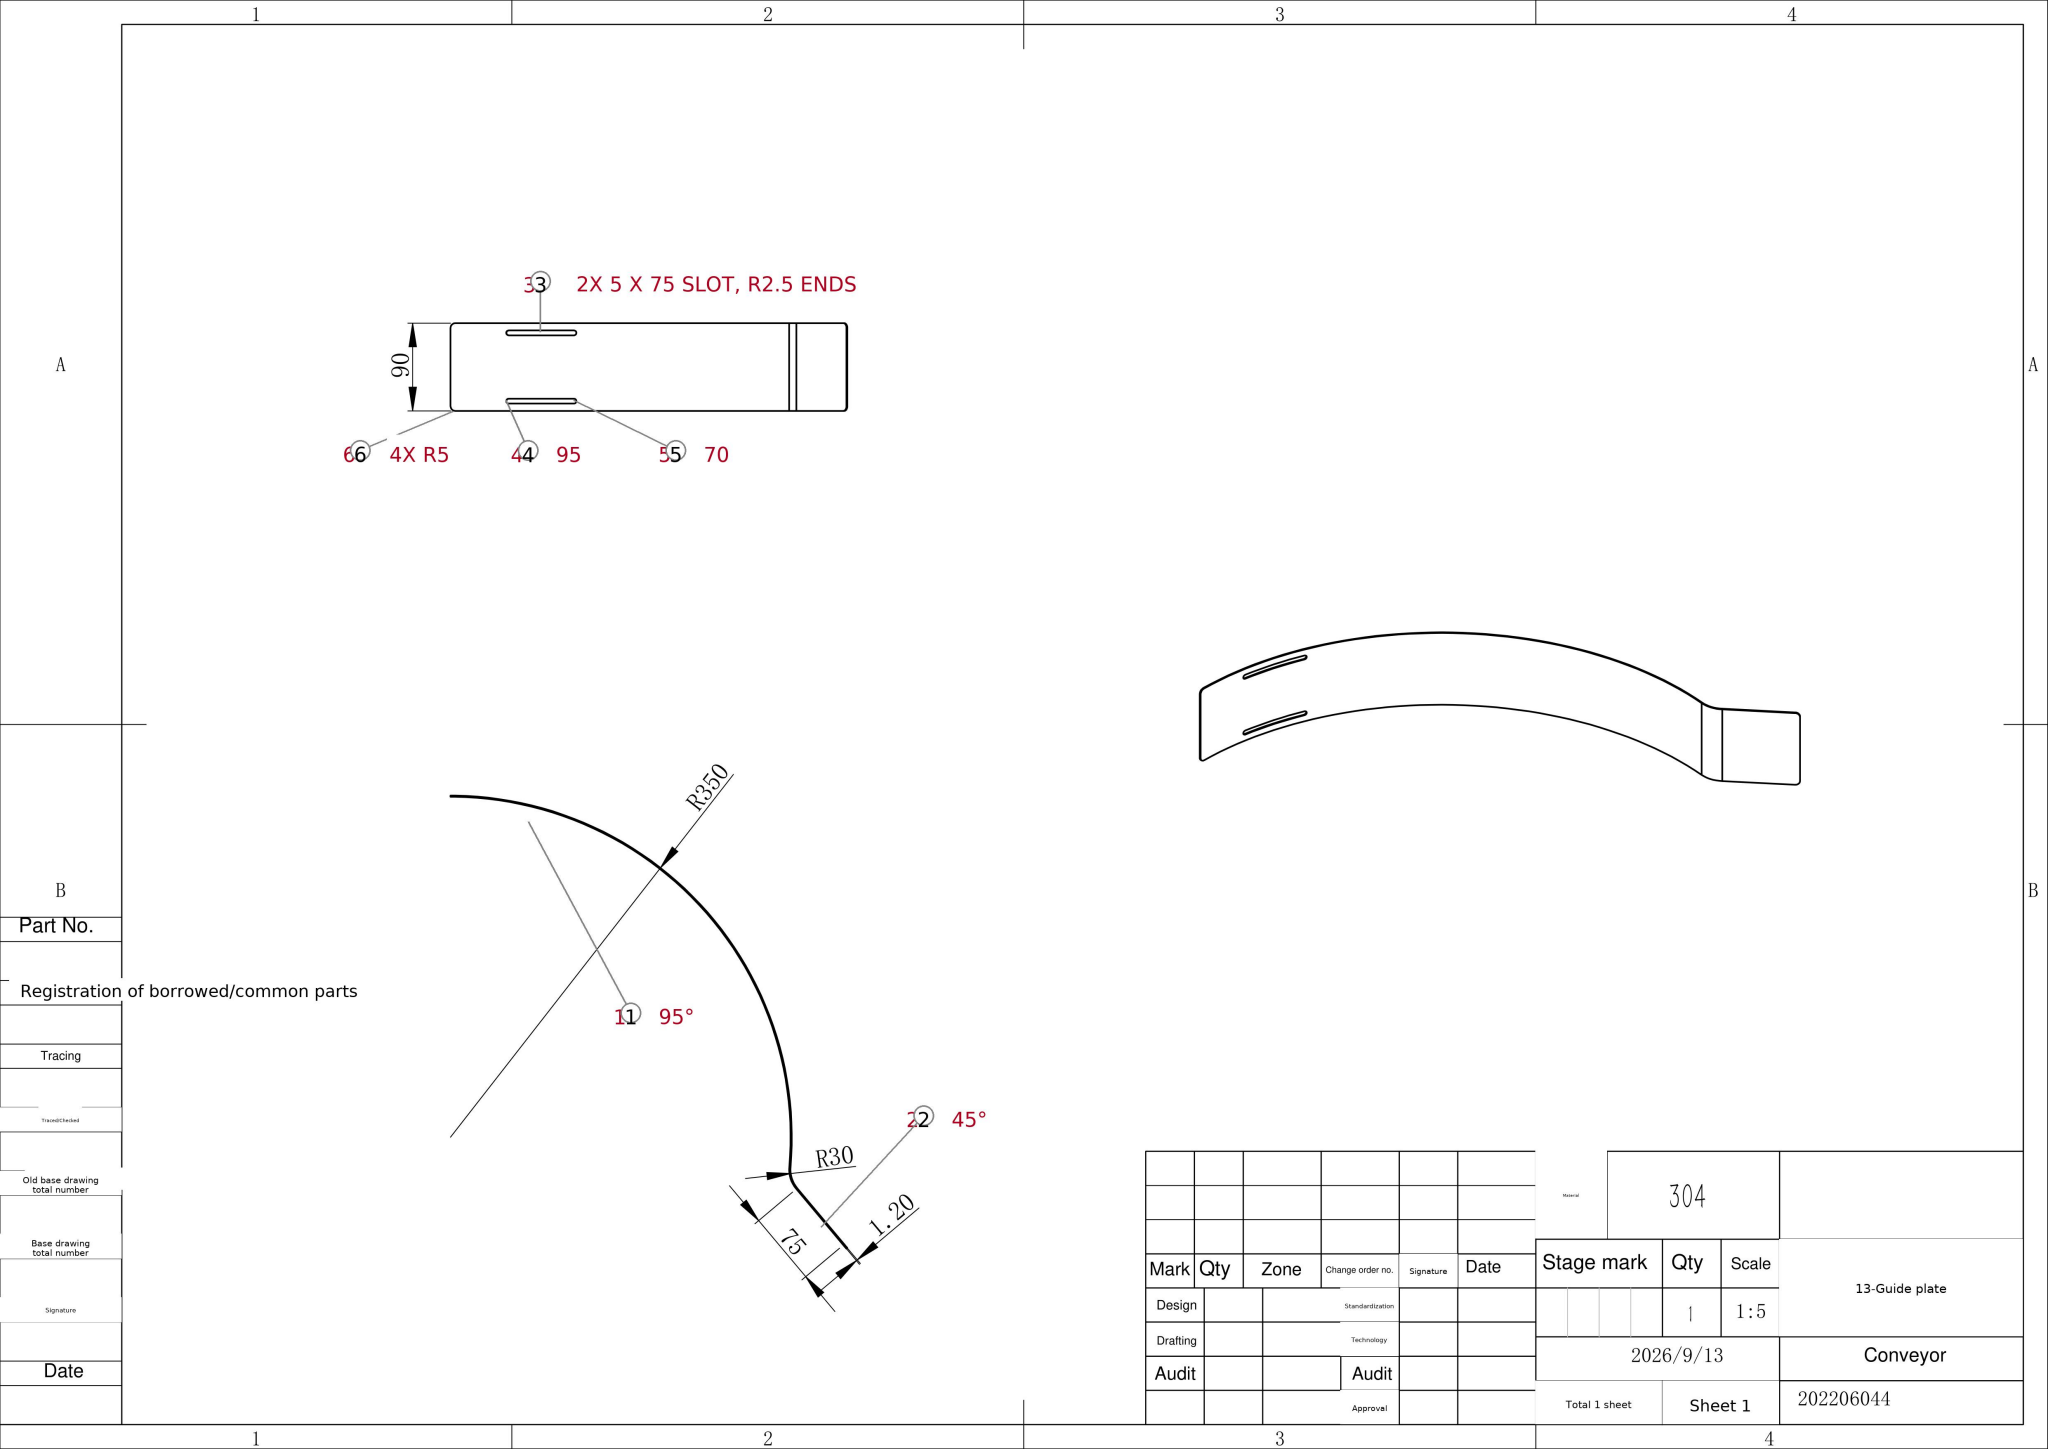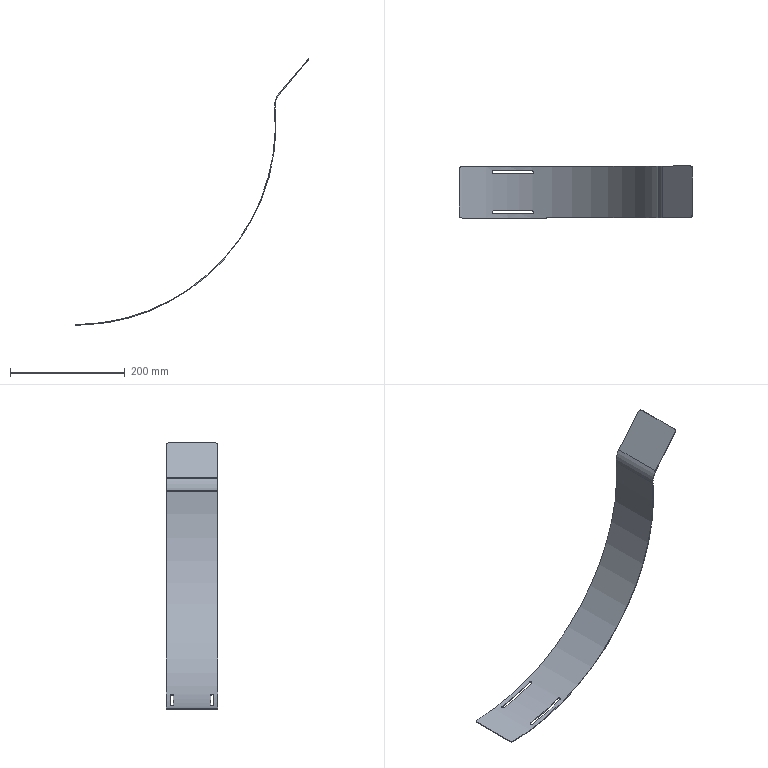Part | SolidWorks | mm | material 304 | 1 solid | 26 faces | box 407 x 90 x 464.46 mm | volume 73026 mm3 | plane 14 | cylinder 8 | spline 4 | commonest cylinder face diameters 10 x4 700 x1 697.6 x1 60 x1 62.4 x1